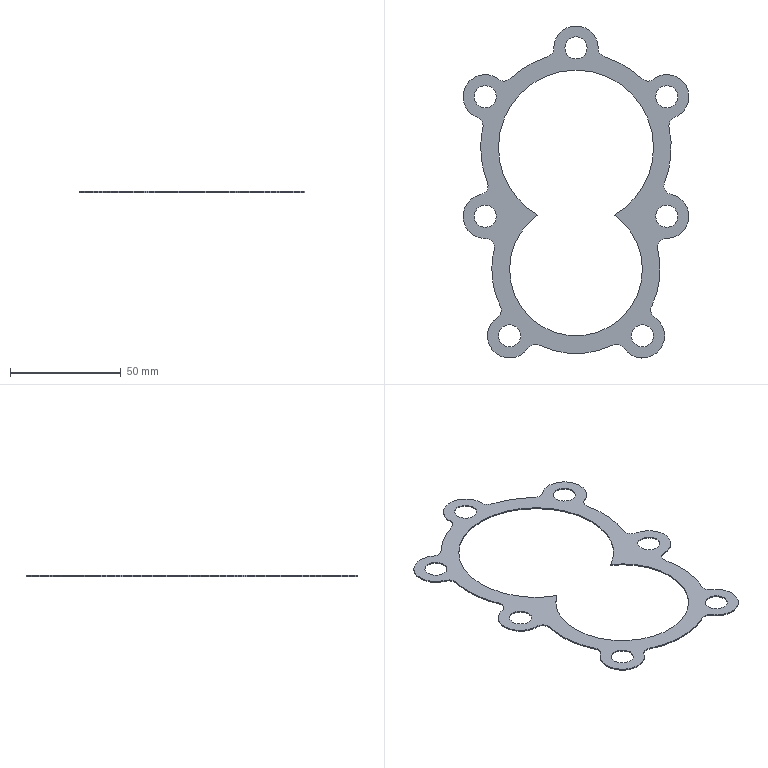Component | SolidWorks | Gasket1-1 | 1 solid | 62 faces | volume 2074 mm3 | cylinder 60 | plane 2 | commonest cylinder face diameters 8 x19 10 x14 20 x12 86 x5 76 x4 70 x3 60 x3